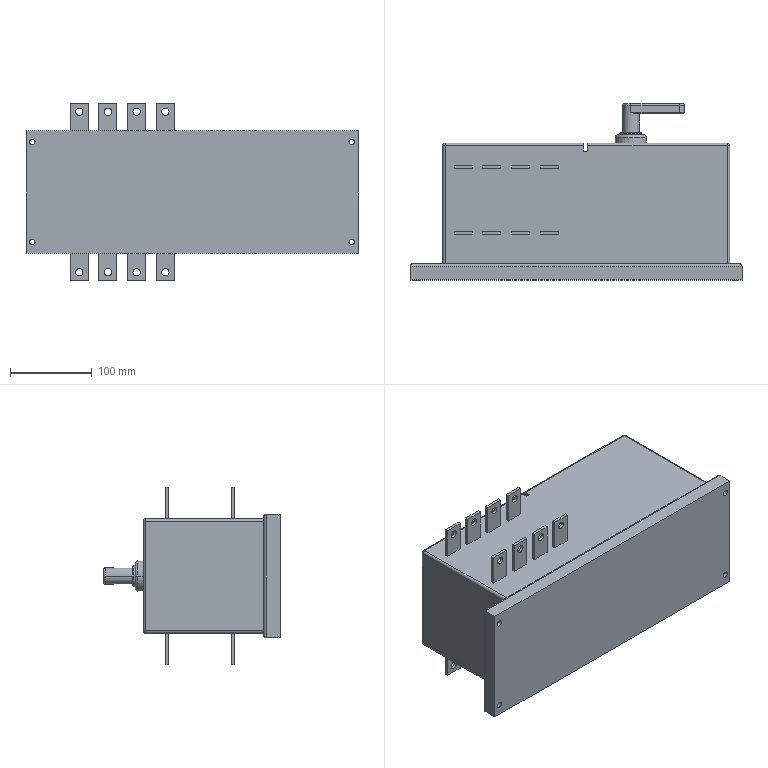Component | SolidWorks | WATSGA-160A-4PCRDualPower-1 | 1 solid | 183 faces | volume 8483220 mm3 | plane 102 | cylinder 68 | torus 9 | sphere 4 | commonest cylinder face diameters 9 x32 6 x14 7 x8 3 x6 20 x2 27 x2 38 x2 12 x2